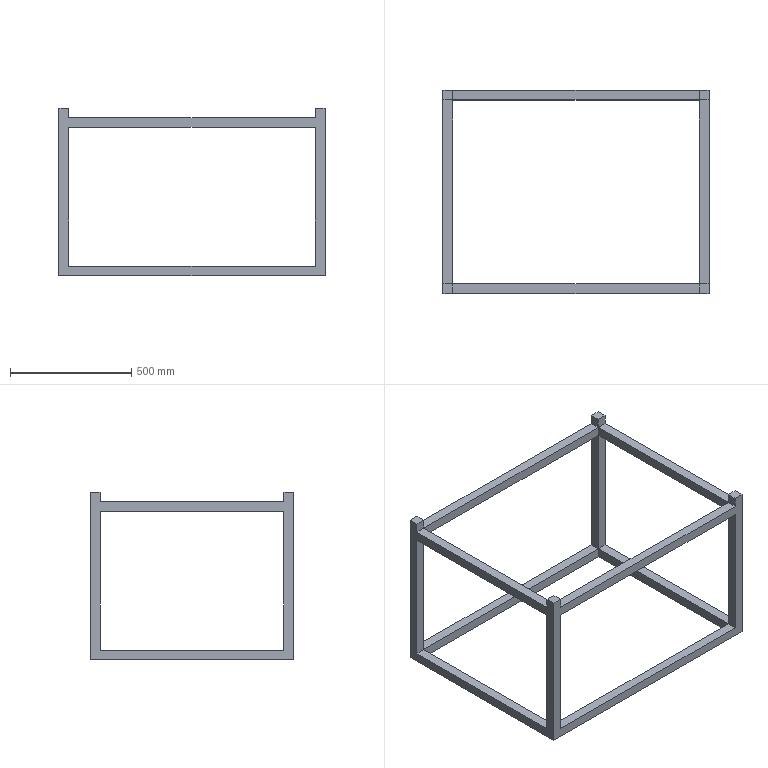Component | SolidWorks | DC-Motor-110-1 | 1 solid | 45 faces | box 1100 x 840 x 694 mm | volume 15833600 mm3 | plane 45
build123d program:
from build123d import *

# Parameters (mm, degrees)
SKETCH1_W           = 1100
SKETCH1_H           = 840
SKETCH1_W_2         = 1020
SKETCH1_H_2         = 760
BOSS_EXTRUDE1_DEPTH = 40
SKETCH2_W           = 40
SKETCH2_H           = 40
BOSS_EXTRUDE2_DEPTH = 574
SKETCH3_W           = 1100
SKETCH3_H           = 840
SKETCH3_W_2         = 1020
SKETCH3_H_2         = 760
BOSS_EXTRUDE3_DEPTH = 40
SKETCH4_W           = 40
SKETCH4_H           = 40
BOSS_EXTRUDE4_DEPTH = 40


with BuildPart() as part:
    # Sketch1 → Boss-Extrude1 (new body)
    with BuildSketch(Plane.XY):
        Rectangle(SKETCH1_W, SKETCH1_H)
        Rectangle(SKETCH1_W_2, SKETCH1_H_2, mode=Mode.SUBTRACT)
    extrude(amount=BOSS_EXTRUDE1_DEPTH)

    # Sketch2 → Boss-Extrude2 (add)
    with BuildSketch(Plane.XY.offset(40)):
        with Locations((-530, 400)):
            Rectangle(SKETCH2_W, SKETCH2_H)
        with Locations((530, 400)):
            Rectangle(SKETCH2_W, SKETCH2_H)
        with Locations((-530, -400)):
            Rectangle(SKETCH2_W, SKETCH2_H)
        with Locations((530, -400)):
            Rectangle(SKETCH2_W, SKETCH2_H)
    extrude(amount=BOSS_EXTRUDE2_DEPTH)

    # Sketch3 → Boss-Extrude3 (add)
    with BuildSketch(Plane.XY.offset(614)):
        Rectangle(SKETCH3_W, SKETCH3_H)
        Rectangle(SKETCH3_W_2, SKETCH3_H_2, mode=Mode.SUBTRACT)
    extrude(amount=BOSS_EXTRUDE3_DEPTH)

    # Sketch4 → Boss-Extrude4 (add)
    with BuildSketch(Plane.XY.offset(654)):
        with Locations((-530, 400)):
            Rectangle(SKETCH4_W, SKETCH4_H)
        with Locations((530, 400)):
            Rectangle(SKETCH4_W, SKETCH4_H)
        with Locations((-530, -400)):
            Rectangle(SKETCH4_W, SKETCH4_H)
        with Locations((530, -400)):
            Rectangle(SKETCH4_W, SKETCH4_H)
    extrude(amount=BOSS_EXTRUDE4_DEPTH)


solid = part.part

# Placed as in the assembly
solid = solid.moved(Location((2.208, 11.801, -420), (0, 0, 0)))